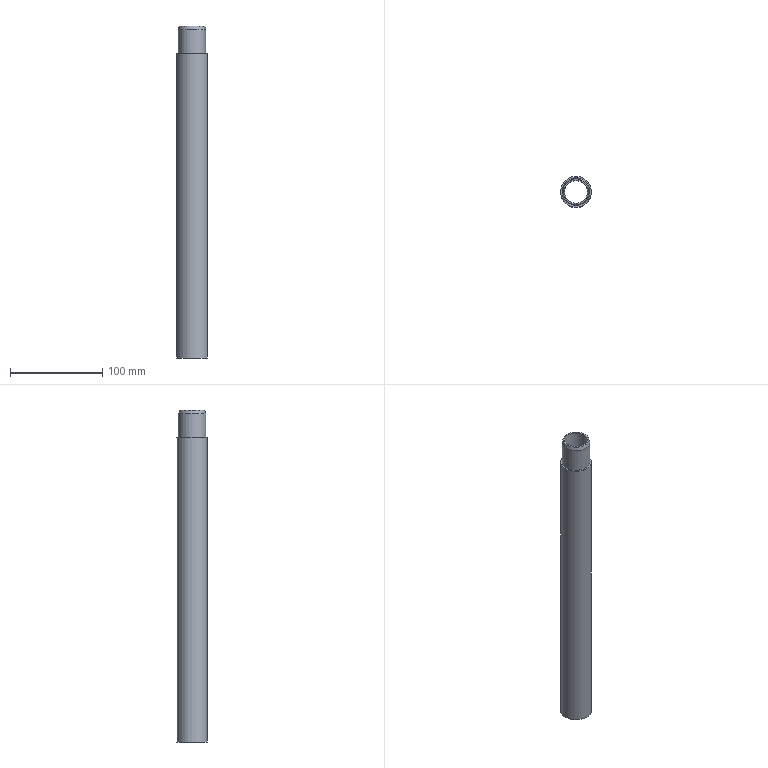Component | NX | CH3404_8_1-2 | 1 solid | 7 faces | box 33.5 x 33.5 x 360 mm | volume 135173 mm3 | plane 3 | cylinder 3 | cone 1 | commonest cylinder face diameters 25 x1 33.5 x1 30 x1
STEP:
#1=CARTESIAN_POINT('',(0.,0.,0.));
#2=DIRECTION('',(0.,0.,1.));
#3=DIRECTION('',(1.,0.,0.));
#4=AXIS2_PLACEMENT_3D('',#1,#2,#3);
#5=CARTESIAN_POINT('',(-12.5,0.,487.));
#6=VERTEX_POINT('',#5);
#7=CARTESIAN_POINT('',(0.,0.,487.));
#8=DIRECTION('',(0.,0.,-1.));
#9=DIRECTION('',(-1.,0.,0.));
#10=AXIS2_PLACEMENT_3D('',#7,#8,#9);
#11=CIRCLE('',#10,12.5);
#12=CARTESIAN_POINT('',(0.,14.,487.));
#13=DIRECTION('',(0.,0.,1.));
#14=DIRECTION('',(1.,0.,0.));
#15=AXIS2_PLACEMENT_3D('',#12,#13,#14);
#16=PLANE('',#15);
#17=CARTESIAN_POINT('',(-12.5,-14.));
#18=CARTESIAN_POINT('',(-12.5,7.651));
#19=CARTESIAN_POINT('',(6.25,-3.175));
#20=CARTESIAN_POINT('',(25.,-14.));
#21=CARTESIAN_POINT('',(6.25,-24.825));
#22=CARTESIAN_POINT('',(-12.5,-35.651));
#23=CARTESIAN_POINT('',(-12.5,-14.));
#24=(BOUNDED_CURVE()B_SPLINE_CURVE(2,(#17,#18,#19,#20,#21,#22,#23),.UNSPECIFIED.,.T.,.F.)B_SPLINE_CURVE_WITH_KNOTS((1,2,2,2,2,1),(-2.094,0.,2.094,4.189,6.283,8.378),.UNSPECIFIED.)CURVE()GEOMETRIC_REPRESENTATION_ITEM()RATIONAL_B_SPLINE_CURVE((1.,0.5,1.,0.5,1.,0.5,1.))REPRESENTATION_ITEM(''));
#25=(GEOMETRIC_REPRESENTATION_CONTEXT(2)PARAMETRIC_REPRESENTATION_CONTEXT()REPRESENTATION_CONTEXT('',''));
#26=DEFINITIONAL_REPRESENTATION('',(#24),#25);
#27=PCURVE('',#16,#26);
#28=CARTESIAN_POINT('',(0.,0.,127.));
#29=DIRECTION('',(0.,0.,-1.));
#30=DIRECTION('',(-1.,0.,0.));
#31=AXIS2_PLACEMENT_3D('',#28,#29,#30);
#32=CYLINDRICAL_SURFACE('',#31,12.5);
#33=CARTESIAN_POINT('',(0.,-360.));
#34=DIRECTION('',(1.,0.));
#35=VECTOR('',#34,1.);
#36=LINE('',#33,#35);
#37=(GEOMETRIC_REPRESENTATION_CONTEXT(2)PARAMETRIC_REPRESENTATION_CONTEXT()REPRESENTATION_CONTEXT('',''));
#38=DEFINITIONAL_REPRESENTATION('',(#36),#37);
#39=PCURVE('',#32,#38);
#40=SURFACE_CURVE('',#11,(#27,#39),.PCURVE_S1.);
#41=EDGE_CURVE('',#6,#6,#40,.T.);
#42=ORIENTED_EDGE('',*,*,#41,.T.);
#43=EDGE_LOOP('',(#42));
#44=FACE_BOUND('',#43,.T.);
#45=CARTESIAN_POINT('',(-14.,0.,487.));
#46=VERTEX_POINT('',#45);
#47=CARTESIAN_POINT('',(0.,0.,487.));
#48=DIRECTION('',(0.,0.,-1.));
#49=DIRECTION('',(-1.,0.,0.));
#50=AXIS2_PLACEMENT_3D('',#47,#48,#49);
#51=CIRCLE('',#50,14.);
#52=CARTESIAN_POINT('',(-14.,-14.));
#53=CARTESIAN_POINT('',(-14.,10.249));
#54=CARTESIAN_POINT('',(7.,-1.876));
#55=CARTESIAN_POINT('',(28.,-14.));
#56=CARTESIAN_POINT('',(7.,-26.124));
#57=CARTESIAN_POINT('',(-14.,-38.249));
#58=CARTESIAN_POINT('',(-14.,-14.));
#59=(BOUNDED_CURVE()B_SPLINE_CURVE(2,(#52,#53,#54,#55,#56,#57,#58),.UNSPECIFIED.,.T.,.F.)B_SPLINE_CURVE_WITH_KNOTS((1,2,2,2,2,1),(-2.094,0.,2.094,4.189,6.283,8.378),.UNSPECIFIED.)CURVE()GEOMETRIC_REPRESENTATION_ITEM()RATIONAL_B_SPLINE_CURVE((1.,0.5,1.,0.5,1.,0.5,1.))REPRESENTATION_ITEM(''));
#60=(GEOMETRIC_REPRESENTATION_CONTEXT(2)PARAMETRIC_REPRESENTATION_CONTEXT()REPRESENTATION_CONTEXT('',''));
#61=DEFINITIONAL_REPRESENTATION('',(#59),#60);
#62=PCURVE('',#16,#61);
#63=CARTESIAN_POINT('',(0.,0.,483.));
#64=DIRECTION('',(0.,0.,-1.));
#65=DIRECTION('',(-1.,0.,0.));
#66=AXIS2_PLACEMENT_3D('',#63,#64,#65);
#67=CONICAL_SURFACE('',#66,15.,0.245);
#68=CARTESIAN_POINT('',(0.,-4.));
#69=DIRECTION('',(1.,0.));
#70=VECTOR('',#69,1.);
#71=LINE('',#68,#70);
#72=(GEOMETRIC_REPRESENTATION_CONTEXT(2)PARAMETRIC_REPRESENTATION_CONTEXT()REPRESENTATION_CONTEXT('',''));
#73=DEFINITIONAL_REPRESENTATION('',(#71),#72);
#74=PCURVE('',#67,#73);
#75=SURFACE_CURVE('',#51,(#62,#74),.PCURVE_S1.);
#76=EDGE_CURVE('',#46,#46,#75,.T.);
#77=ORIENTED_EDGE('',*,*,#76,.F.);
#78=EDGE_LOOP('',(#77));
#79=FACE_BOUND('',#78,.T.);
#80=ADVANCED_FACE('',(#44,#79),#16,.T.);
#81=CARTESIAN_POINT('',(-12.5,0.,127.));
#82=VERTEX_POINT('',#81);
#83=CARTESIAN_POINT('',(0.,0.,127.));
#84=DIRECTION('',(0.,0.,-1.));
#85=DIRECTION('',(-1.,0.,0.));
#86=AXIS2_PLACEMENT_3D('',#83,#84,#85);
#87=CIRCLE('',#86,12.5);
#88=CARTESIAN_POINT('',(0.,0.));
#89=DIRECTION('',(1.,0.));
#90=VECTOR('',#89,1.);
#91=LINE('',#88,#90);
#92=(GEOMETRIC_REPRESENTATION_CONTEXT(2)PARAMETRIC_REPRESENTATION_CONTEXT()REPRESENTATION_CONTEXT('',''));
#93=DEFINITIONAL_REPRESENTATION('',(#91),#92);
#94=PCURVE('',#32,#93);
#95=CARTESIAN_POINT('',(0.,12.5,127.));
#96=DIRECTION('',(0.,0.,-1.));
#97=DIRECTION('',(-1.,0.,0.));
#98=AXIS2_PLACEMENT_3D('',#95,#96,#97);
#99=PLANE('',#98);
#100=CARTESIAN_POINT('',(0.,-12.5));
#101=DIRECTION('',(1.,0.));
#102=AXIS2_PLACEMENT_2D('',#100,#101);
#103=CIRCLE('',#102,12.5);
#104=(GEOMETRIC_REPRESENTATION_CONTEXT(2)PARAMETRIC_REPRESENTATION_CONTEXT()REPRESENTATION_CONTEXT('',''));
#105=DEFINITIONAL_REPRESENTATION('',(#103),#104);
#106=PCURVE('',#99,#105);
#107=SURFACE_CURVE('',#87,(#94,#106),.PCURVE_S1.);
#108=EDGE_CURVE('',#82,#82,#107,.T.);
#109=ORIENTED_EDGE('',*,*,#108,.F.);
#110=CARTESIAN_POINT('',(-12.5,-0.,487.));
#111=CARTESIAN_POINT('',(-12.5,-0.,127.));
#112=B_SPLINE_CURVE_WITH_KNOTS('',1,(#110,#111),.UNSPECIFIED.,.F.,.F.,(2,2),(-360.,0.),.PIECEWISE_BEZIER_KNOTS.);
#113=CARTESIAN_POINT('',(0.,0.));
#114=DIRECTION('',(0.,1.));
#115=VECTOR('',#114,1.);
#116=LINE('',#113,#115);
#117=(GEOMETRIC_REPRESENTATION_CONTEXT(2)PARAMETRIC_REPRESENTATION_CONTEXT()REPRESENTATION_CONTEXT('',''));
#118=DEFINITIONAL_REPRESENTATION('',(#116),#117);
#119=PCURVE('',#32,#118);
#120=CARTESIAN_POINT('',(6.283,0.));
#121=DIRECTION('',(0.,1.));
#122=VECTOR('',#121,1.);
#123=LINE('',#120,#122);
#124=(GEOMETRIC_REPRESENTATION_CONTEXT(2)PARAMETRIC_REPRESENTATION_CONTEXT()REPRESENTATION_CONTEXT('',''));
#125=DEFINITIONAL_REPRESENTATION('',(#123),#124);
#126=PCURVE('',#32,#125);
#127=SEAM_CURVE('',#112,(#119,#126),.PCURVE_S1.);
#128=EDGE_CURVE('',#6,#82,#127,.T.);
#129=ORIENTED_EDGE('',*,*,#128,.F.);
#130=ORIENTED_EDGE('',*,*,#41,.T.);
#131=ORIENTED_EDGE('',*,*,#128,.T.);
#132=EDGE_LOOP('',(#109,#129,#130,#131));
#133=FACE_BOUND('',#132,.F.);
#134=ADVANCED_FACE('',(#133),#32,.F.);
#135=CARTESIAN_POINT('',(-16.75,0.,127.));
#136=VERTEX_POINT('',#135);
#137=CARTESIAN_POINT('',(0.,0.,127.));
#138=DIRECTION('',(0.,0.,-1.));
#139=DIRECTION('',(-1.,0.,0.));
#140=AXIS2_PLACEMENT_3D('',#137,#138,#139);
#141=CIRCLE('',#140,16.75);
#142=CARTESIAN_POINT('',(0.,-12.5));
#143=DIRECTION('',(1.,0.));
#144=AXIS2_PLACEMENT_2D('',#142,#143);
#145=CIRCLE('',#144,16.75);
#146=(GEOMETRIC_REPRESENTATION_CONTEXT(2)PARAMETRIC_REPRESENTATION_CONTEXT()REPRESENTATION_CONTEXT('',''));
#147=DEFINITIONAL_REPRESENTATION('',(#145),#146);
#148=PCURVE('',#99,#147);
#149=CARTESIAN_POINT('',(0.,0.,127.));
#150=DIRECTION('',(0.,0.,-1.));
#151=DIRECTION('',(-1.,0.,0.));
#152=AXIS2_PLACEMENT_3D('',#149,#150,#151);
#153=CYLINDRICAL_SURFACE('',#152,16.75);
#154=CARTESIAN_POINT('',(0.,0.));
#155=DIRECTION('',(1.,0.));
#156=VECTOR('',#155,1.);
#157=LINE('',#154,#156);
#158=(GEOMETRIC_REPRESENTATION_CONTEXT(2)PARAMETRIC_REPRESENTATION_CONTEXT()REPRESENTATION_CONTEXT('',''));
#159=DEFINITIONAL_REPRESENTATION('',(#157),#158);
#160=PCURVE('',#153,#159);
#161=SURFACE_CURVE('',#141,(#148,#160),.PCURVE_S1.);
#162=EDGE_CURVE('',#136,#136,#161,.T.);
#163=ORIENTED_EDGE('',*,*,#162,.T.);
#164=EDGE_LOOP('',(#163));
#165=FACE_BOUND('',#164,.T.);
#166=ORIENTED_EDGE('',*,*,#108,.F.);
#167=EDGE_LOOP('',(#166));
#168=FACE_BOUND('',#167,.T.);
#169=ADVANCED_FACE('',(#165,#168),#99,.T.);
#170=CARTESIAN_POINT('',(-16.75,0.,457.));
#171=VERTEX_POINT('',#170);
#172=CARTESIAN_POINT('',(0.,0.,457.));
#173=DIRECTION('',(0.,0.,-1.));
#174=DIRECTION('',(-1.,0.,0.));
#175=AXIS2_PLACEMENT_3D('',#172,#173,#174);
#176=CIRCLE('',#175,16.75);
#177=CARTESIAN_POINT('',(0.,-330.));
#178=DIRECTION('',(1.,0.));
#179=VECTOR('',#178,1.);
#180=LINE('',#177,#179);
#181=(GEOMETRIC_REPRESENTATION_CONTEXT(2)PARAMETRIC_REPRESENTATION_CONTEXT()REPRESENTATION_CONTEXT('',''));
#182=DEFINITIONAL_REPRESENTATION('',(#180),#181);
#183=PCURVE('',#153,#182);
#184=CARTESIAN_POINT('',(0.,16.75,457.));
#185=DIRECTION('',(0.,0.,1.));
#186=DIRECTION('',(1.,0.,0.));
#187=AXIS2_PLACEMENT_3D('',#184,#185,#186);
#188=PLANE('',#187);
#189=CARTESIAN_POINT('',(-16.75,-16.75));
#190=CARTESIAN_POINT('',(-16.75,12.262));
#191=CARTESIAN_POINT('',(8.375,-2.244));
#192=CARTESIAN_POINT('',(33.5,-16.75));
#193=CARTESIAN_POINT('',(8.375,-31.256));
#194=CARTESIAN_POINT('',(-16.75,-45.762));
#195=CARTESIAN_POINT('',(-16.75,-16.75));
#196=(BOUNDED_CURVE()B_SPLINE_CURVE(2,(#189,#190,#191,#192,#193,#194,#195),.UNSPECIFIED.,.T.,.F.)B_SPLINE_CURVE_WITH_KNOTS((1,2,2,2,2,1),(-2.094,0.,2.094,4.189,6.283,8.378),.UNSPECIFIED.)CURVE()GEOMETRIC_REPRESENTATION_ITEM()RATIONAL_B_SPLINE_CURVE((1.,0.5,1.,0.5,1.,0.5,1.))REPRESENTATION_ITEM(''));
#197=(GEOMETRIC_REPRESENTATION_CONTEXT(2)PARAMETRIC_REPRESENTATION_CONTEXT()REPRESENTATION_CONTEXT('',''));
#198=DEFINITIONAL_REPRESENTATION('',(#196),#197);
#199=PCURVE('',#188,#198);
#200=SURFACE_CURVE('',#176,(#183,#199),.PCURVE_S1.);
#201=EDGE_CURVE('',#171,#171,#200,.T.);
#202=ORIENTED_EDGE('',*,*,#201,.T.);
#203=CARTESIAN_POINT('',(-16.75,0.,457.));
#204=CARTESIAN_POINT('',(-16.75,0.,127.));
#205=B_SPLINE_CURVE_WITH_KNOTS('',1,(#203,#204),.UNSPECIFIED.,.F.,.F.,(2,2),(-330.,0.),.PIECEWISE_BEZIER_KNOTS.);
#206=CARTESIAN_POINT('',(6.283,0.));
#207=DIRECTION('',(0.,1.));
#208=VECTOR('',#207,1.);
#209=LINE('',#206,#208);
#210=(GEOMETRIC_REPRESENTATION_CONTEXT(2)PARAMETRIC_REPRESENTATION_CONTEXT()REPRESENTATION_CONTEXT('',''));
#211=DEFINITIONAL_REPRESENTATION('',(#209),#210);
#212=PCURVE('',#153,#211);
#213=CARTESIAN_POINT('',(0.,0.));
#214=DIRECTION('',(0.,1.));
#215=VECTOR('',#214,1.);
#216=LINE('',#213,#215);
#217=(GEOMETRIC_REPRESENTATION_CONTEXT(2)PARAMETRIC_REPRESENTATION_CONTEXT()REPRESENTATION_CONTEXT('',''));
#218=DEFINITIONAL_REPRESENTATION('',(#216),#217);
#219=PCURVE('',#153,#218);
#220=SEAM_CURVE('',#205,(#212,#219),.PCURVE_S1.);
#221=EDGE_CURVE('',#171,#136,#220,.T.);
#222=ORIENTED_EDGE('',*,*,#221,.T.);
#223=ORIENTED_EDGE('',*,*,#162,.F.);
#224=ORIENTED_EDGE('',*,*,#221,.F.);
#225=EDGE_LOOP('',(#202,#222,#223,#224));
#226=FACE_BOUND('',#225,.T.);
#227=ADVANCED_FACE('',(#226),#153,.T.);
#228=CARTESIAN_POINT('',(-15.,0.,457.));
#229=VERTEX_POINT('',#228);
#230=CARTESIAN_POINT('',(0.,0.,457.));
#231=DIRECTION('',(0.,0.,-1.));
#232=DIRECTION('',(-1.,0.,0.));
#233=AXIS2_PLACEMENT_3D('',#230,#231,#232);
#234=CIRCLE('',#233,15.);
#235=CARTESIAN_POINT('',(-15.,-16.75));
#236=CARTESIAN_POINT('',(-15.,9.231));
#237=CARTESIAN_POINT('',(7.5,-3.76));
#238=CARTESIAN_POINT('',(30.,-16.75));
#239=CARTESIAN_POINT('',(7.5,-29.74));
#240=CARTESIAN_POINT('',(-15.,-42.731));
#241=CARTESIAN_POINT('',(-15.,-16.75));
#242=(BOUNDED_CURVE()B_SPLINE_CURVE(2,(#235,#236,#237,#238,#239,#240,#241),.UNSPECIFIED.,.T.,.F.)B_SPLINE_CURVE_WITH_KNOTS((1,2,2,2,2,1),(-2.094,0.,2.094,4.189,6.283,8.378),.UNSPECIFIED.)CURVE()GEOMETRIC_REPRESENTATION_ITEM()RATIONAL_B_SPLINE_CURVE((1.,0.5,1.,0.5,1.,0.5,1.))REPRESENTATION_ITEM(''));
#243=(GEOMETRIC_REPRESENTATION_CONTEXT(2)PARAMETRIC_REPRESENTATION_CONTEXT()REPRESENTATION_CONTEXT('',''));
#244=DEFINITIONAL_REPRESENTATION('',(#242),#243);
#245=PCURVE('',#188,#244);
#246=CARTESIAN_POINT('',(0.,0.,127.));
#247=DIRECTION('',(0.,0.,-1.));
#248=DIRECTION('',(-1.,0.,0.));
#249=AXIS2_PLACEMENT_3D('',#246,#247,#248);
#250=CYLINDRICAL_SURFACE('',#249,15.);
#251=CARTESIAN_POINT('',(0.,-330.));
#252=DIRECTION('',(1.,0.));
#253=VECTOR('',#252,1.);
#254=LINE('',#251,#253);
#255=(GEOMETRIC_REPRESENTATION_CONTEXT(2)PARAMETRIC_REPRESENTATION_CONTEXT()REPRESENTATION_CONTEXT('',''));
#256=DEFINITIONAL_REPRESENTATION('',(#254),#255);
#257=PCURVE('',#250,#256);
#258=SURFACE_CURVE('',#234,(#245,#257),.PCURVE_S1.);
#259=EDGE_CURVE('',#229,#229,#258,.T.);
#260=ORIENTED_EDGE('',*,*,#259,.T.);
#261=EDGE_LOOP('',(#260));
#262=FACE_BOUND('',#261,.T.);
#263=ORIENTED_EDGE('',*,*,#201,.F.);
#264=EDGE_LOOP('',(#263));
#265=FACE_BOUND('',#264,.T.);
#266=ADVANCED_FACE('',(#262,#265),#188,.T.);
#267=CARTESIAN_POINT('',(-15.,0.,483.));
#268=VERTEX_POINT('',#267);
#269=CARTESIAN_POINT('',(0.,0.,483.));
#270=DIRECTION('',(0.,0.,-1.));
#271=DIRECTION('',(-1.,0.,0.));
#272=AXIS2_PLACEMENT_3D('',#269,#270,#271);
#273=CIRCLE('',#272,15.);
#274=CARTESIAN_POINT('',(0.,-356.));
#275=DIRECTION('',(1.,0.));
#276=VECTOR('',#275,1.);
#277=LINE('',#274,#276);
#278=(GEOMETRIC_REPRESENTATION_CONTEXT(2)PARAMETRIC_REPRESENTATION_CONTEXT()REPRESENTATION_CONTEXT('',''));
#279=DEFINITIONAL_REPRESENTATION('',(#277),#278);
#280=PCURVE('',#250,#279);
#281=CARTESIAN_POINT('',(0.,0.));
#282=DIRECTION('',(1.,0.));
#283=VECTOR('',#282,1.);
#284=LINE('',#281,#283);
#285=(GEOMETRIC_REPRESENTATION_CONTEXT(2)PARAMETRIC_REPRESENTATION_CONTEXT()REPRESENTATION_CONTEXT('',''));
#286=DEFINITIONAL_REPRESENTATION('',(#284),#285);
#287=PCURVE('',#67,#286);
#288=SURFACE_CURVE('',#273,(#280,#287),.PCURVE_S1.);
#289=EDGE_CURVE('',#268,#268,#288,.T.);
#290=ORIENTED_EDGE('',*,*,#289,.T.);
#291=CARTESIAN_POINT('',(-15.,0.,483.));
#292=CARTESIAN_POINT('',(-15.,0.,457.));
#293=B_SPLINE_CURVE_WITH_KNOTS('',1,(#291,#292),.UNSPECIFIED.,.F.,.F.,(2,2),(-356.,-330.),.PIECEWISE_BEZIER_KNOTS.);
#294=CARTESIAN_POINT('',(6.283,0.));
#295=DIRECTION('',(0.,1.));
#296=VECTOR('',#295,1.);
#297=LINE('',#294,#296);
#298=(GEOMETRIC_REPRESENTATION_CONTEXT(2)PARAMETRIC_REPRESENTATION_CONTEXT()REPRESENTATION_CONTEXT('',''));
#299=DEFINITIONAL_REPRESENTATION('',(#297),#298);
#300=PCURVE('',#250,#299);
#301=CARTESIAN_POINT('',(0.,0.));
#302=DIRECTION('',(0.,1.));
#303=VECTOR('',#302,1.);
#304=LINE('',#301,#303);
#305=(GEOMETRIC_REPRESENTATION_CONTEXT(2)PARAMETRIC_REPRESENTATION_CONTEXT()REPRESENTATION_CONTEXT('',''));
#306=DEFINITIONAL_REPRESENTATION('',(#304),#305);
#307=PCURVE('',#250,#306);
#308=SEAM_CURVE('',#293,(#300,#307),.PCURVE_S1.);
#309=EDGE_CURVE('',#268,#229,#308,.T.);
#310=ORIENTED_EDGE('',*,*,#309,.T.);
#311=ORIENTED_EDGE('',*,*,#259,.F.);
#312=ORIENTED_EDGE('',*,*,#309,.F.);
#313=EDGE_LOOP('',(#290,#310,#311,#312));
#314=FACE_BOUND('',#313,.T.);
#315=ADVANCED_FACE('',(#314),#250,.T.);
#316=ORIENTED_EDGE('',*,*,#76,.T.);
#317=CARTESIAN_POINT('',(-14.,0.,487.));
#318=CARTESIAN_POINT('',(-15.,0.,483.));
#319=B_SPLINE_CURVE_WITH_KNOTS('',1,(#317,#318),.UNSPECIFIED.,.F.,.F.,(2,2),(-4.123,0.),.PIECEWISE_BEZIER_KNOTS.);
#320=CARTESIAN_POINT('',(6.283,0.));
#321=DIRECTION('',(0.,1.));
#322=VECTOR('',#321,1.);
#323=LINE('',#320,#322);
#324=(GEOMETRIC_REPRESENTATION_CONTEXT(2)PARAMETRIC_REPRESENTATION_CONTEXT()REPRESENTATION_CONTEXT('',''));
#325=DEFINITIONAL_REPRESENTATION('',(#323),#324);
#326=PCURVE('',#67,#325);
#327=CARTESIAN_POINT('',(0.,0.));
#328=DIRECTION('',(0.,1.));
#329=VECTOR('',#328,1.);
#330=LINE('',#327,#329);
#331=(GEOMETRIC_REPRESENTATION_CONTEXT(2)PARAMETRIC_REPRESENTATION_CONTEXT()REPRESENTATION_CONTEXT('',''));
#332=DEFINITIONAL_REPRESENTATION('',(#330),#331);
#333=PCURVE('',#67,#332);
#334=SEAM_CURVE('',#319,(#326,#333),.PCURVE_S1.);
#335=EDGE_CURVE('',#46,#268,#334,.T.);
#336=ORIENTED_EDGE('',*,*,#335,.T.);
#337=ORIENTED_EDGE('',*,*,#289,.F.);
#338=ORIENTED_EDGE('',*,*,#335,.F.);
#339=EDGE_LOOP('',(#316,#336,#337,#338));
#340=FACE_BOUND('',#339,.T.);
#341=ADVANCED_FACE('',(#340),#67,.T.);
#342=CLOSED_SHELL('',(#80,#134,#169,#227,#266,#315,#341));
#343=MANIFOLD_SOLID_BREP('',#342);
#344=(LENGTH_UNIT()NAMED_UNIT(*)SI_UNIT(.MILLI.,.METRE.));
#345=UNCERTAINTY_MEASURE_WITH_UNIT(LENGTH_MEASURE(0.00001),#344,'','');
#346=(NAMED_UNIT(*)PLANE_ANGLE_UNIT()SI_UNIT($,.RADIAN.));
#347=(NAMED_UNIT(*)SI_UNIT($,.STERADIAN.)SOLID_ANGLE_UNIT());
#348=(GEOMETRIC_REPRESENTATION_CONTEXT(3)GLOBAL_UNCERTAINTY_ASSIGNED_CONTEXT((#345))GLOBAL_UNIT_ASSIGNED_CONTEXT((#344,#346,#347))REPRESENTATION_CONTEXT('',''));
#349=ADVANCED_BREP_SHAPE_REPRESENTATION('',(#4,#343),#348);